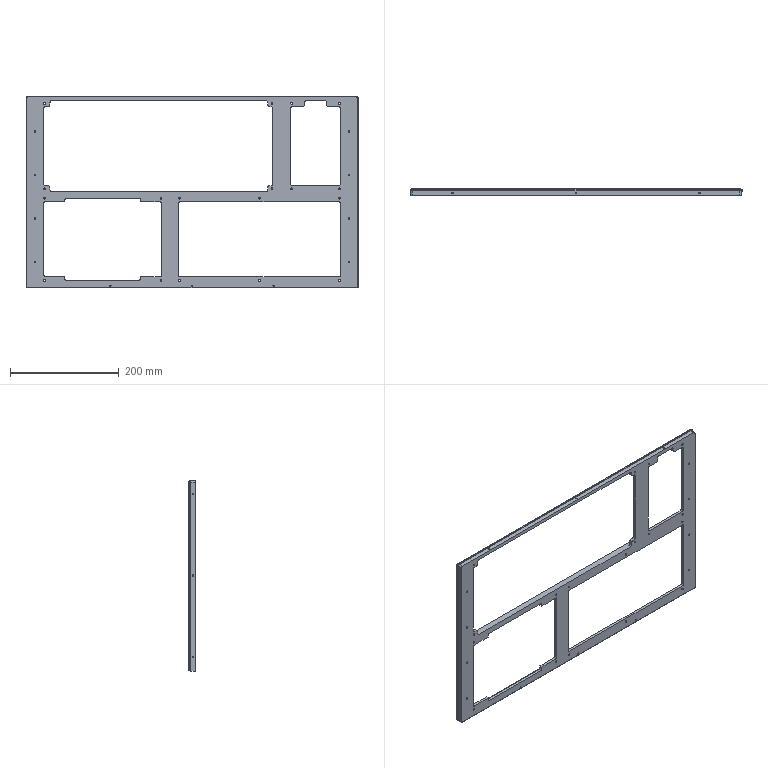CAM job | Mastercam | mm | 15 operations | part box 610 x 12 x 352.46
1. Drill/Counterbore | 7 - 4 倒角刀
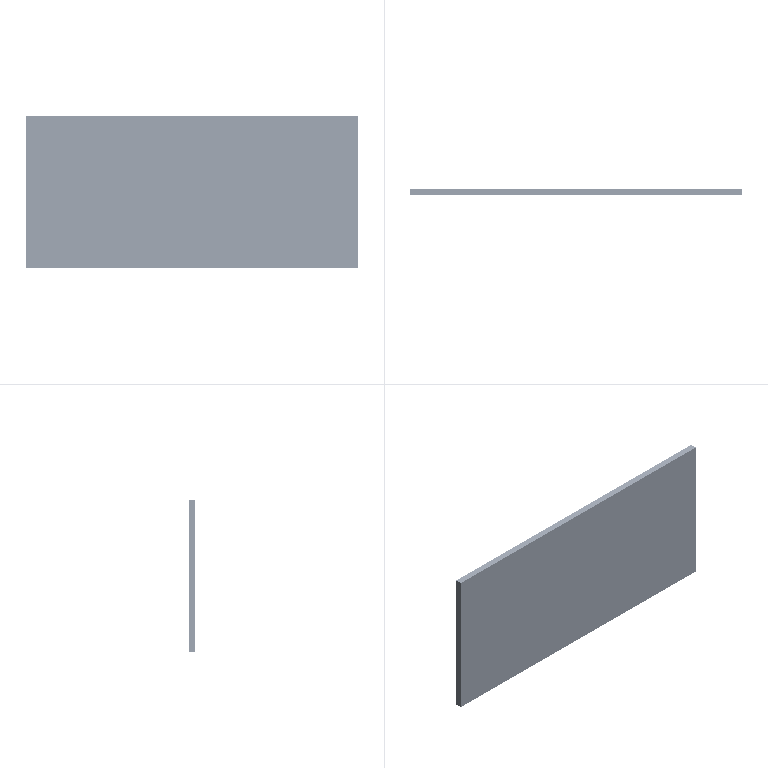2. Drill/Counterbore | 7 - 4 倒角刀
3. Peck Drill | 1 - 2.5 钻头
4. Drill/Counterbore | 7 - 4 倒角刀
5. Peck Drill | 1 - 2.5 钻头
6. Drill/Counterbore | 7 - 4 倒角刀
7. Peck Drill | 1 - 2.5 钻头
8. Drill/Counterbore | 7 - 4 倒角刀
9. Peck Drill | 1 - 2.5 钻头
10. Drill/Counterbore | 7 - 4 倒角刀
11. Peck Drill | 1 - 2.5 钻头
12. Drill/Counterbore | 7 - 4 倒角刀
13. Peck Drill | 1 - 2.5 钻头
14. Drill/Counterbore | 7 - 4 倒角刀
15. Peck Drill | 1 - 2.5 钻头